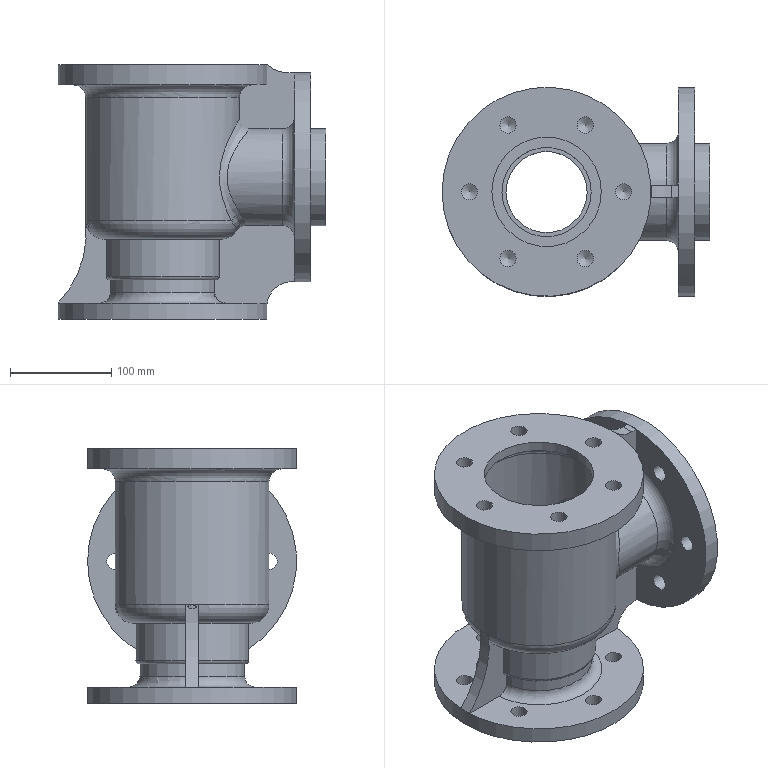Component | NX | 01__BODY__2 | 4 solids | 101 faces | volume 2711777 mm3 | cylinder 42 | plane 31 | torus 16 | spline 6 | cone 6 | commonest cylinder face diameters 16 x18 96 x4 206 x4 112 x3 104 x3 152 x2 128 x1 108 x1